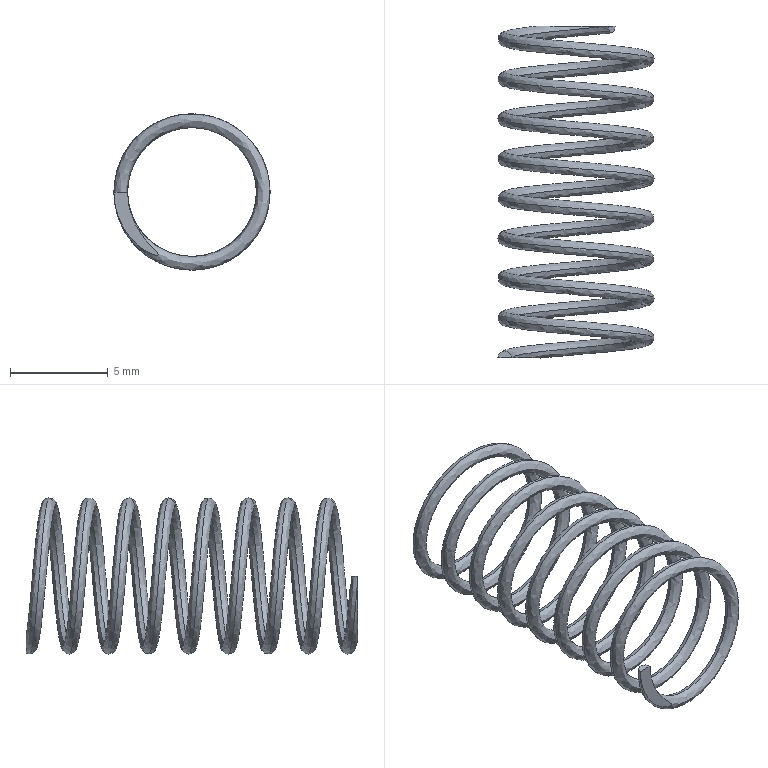Component | SolidWorks | YWF-D8-L25CompressionSpring-1 | 1 solid | 6 faces | volume 73 mm3 | plane 4 | spline 2